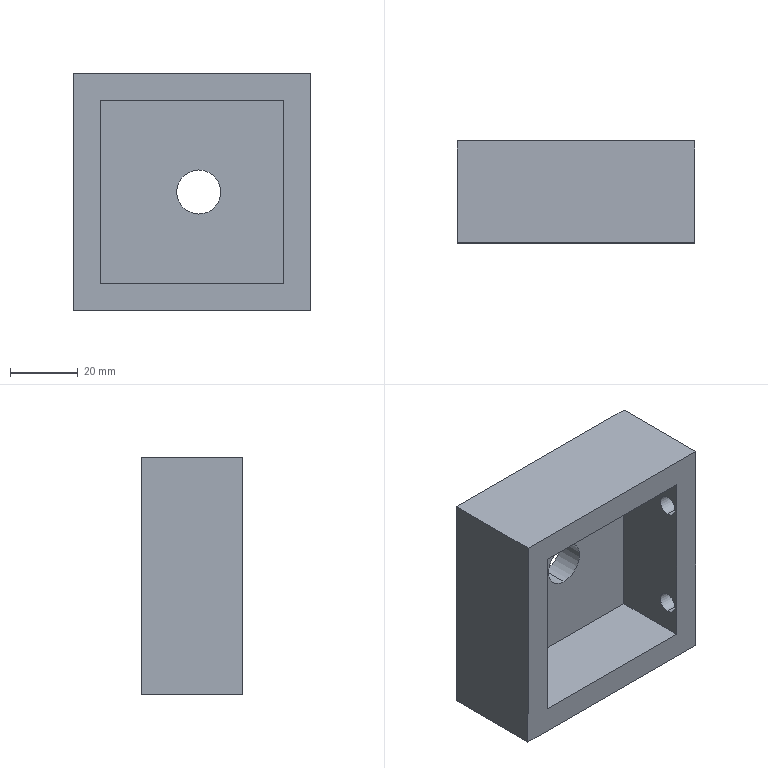Component | SolidWorks | GrippingMountingHousing-2 | 1 solid | 17 faces | box 70.08 x 30 x 70.08 mm | volume 81334 mm3 | plane 11 | cylinder 6 | commonest cylinder face diameters 6 x4 13 x2
build123d program:
from build123d import *

# Parameters (mm, degrees)
SKETCH1_2_W                   = 30
SKETCH1_2_H                   = 70
BOSS_EXTRUDE1_DEPTH           = 70
SHELL1_T                      = -8
SKETCH4_R                     = 3
CUT_EXTRUDE2_DEPTH            = 10
SKETCH1_R                     = 6.5
PISTON_ROD_THROUGH_HOLE_DEPTH = 8.5


with BuildPart() as part:
    # Sketch1_2 → Boss-Extrude1 (new body)
    with BuildSketch(Plane(origin=(0, 0, 0), x_dir=(1, 0, 0), z_dir=(0, 1, 0))):
        Rectangle(SKETCH1_2_W, SKETCH1_2_H)
    extrude(amount=BOSS_EXTRUDE1_DEPTH)

    # Shell1
    shell1_openings = [part.faces().sort_by_distance(p)[0] for p in [
        (15, 35, 0),
    ]]
    offset(amount=SHELL1_T, openings=shell1_openings, kind=Kind.INTERSECTION)

    # Sketch4 → Cut-Extrude2 (cut)
    with BuildSketch(Plane(origin=(0, 70, 0), x_dir=(1, 0, 0), z_dir=(0, 1, 0))):
        with Locations(Location((11.231, -17.525, 0), (0, 0, 270))):
            Circle(SKETCH4_R)
        with Locations(Location((11.231, 17.525, 0), (0, 0, 270))):
            Circle(SKETCH4_R)
    extrude(amount=-CUT_EXTRUDE2_DEPTH, mode=Mode.SUBTRACT)

    # Sketch1 → Piston Rod Through Hole (cut)
    with BuildSketch(Plane.ZY.offset(15)):
        with Locations((-0.0026, 37.002)):
            Circle(SKETCH1_R)
    extrude(amount=-PISTON_ROD_THROUGH_HOLE_DEPTH, mode=Mode.SUBTRACT)


solid = part.part

# Placed as in the assembly
solid = solid.moved(Location((-162.042, 776.54, 1109.793), (0, 0.0619, -90)))
STEP:
#1=COLOUR_RGB('',0.7922,0.8196,0.9333);
#2=FILL_AREA_STYLE_COLOUR('',#1);
#3=FILL_AREA_STYLE('',(#2));
#4=SURFACE_STYLE_FILL_AREA(#3);
#5=SURFACE_SIDE_STYLE('',(#4));
#6=SURFACE_STYLE_USAGE(.BOTH.,#5);
#7=PRESENTATION_STYLE_ASSIGNMENT((#6));
#8=CARTESIAN_POINT('',(-4.923,30.848,43.947));
#9=VERTEX_POINT('',#8);
#10=CARTESIAN_POINT('',(-4.923,30.848,43.435));
#11=VERTEX_POINT('',#10);
#12=CARTESIAN_POINT('',(-4.923,30.848,43.691));
#13=DIRECTION('',(0.,-1.,0.));
#14=DIRECTION('',(-0.00108,0.,-1.));
#15=AXIS2_PLACEMENT_3D('',#12,#13,#14);
#16=CIRCLE('',#15,0.2559);
#17=EDGE_CURVE('',#9,#11,#16,.T.);
#18=ORIENTED_EDGE('',*,*,#17,.T.);
#19=CARTESIAN_POINT('',(-4.923,31.163,43.435));
#20=VERTEX_POINT('',#19);
#21=CARTESIAN_POINT('',(-4.923,30.828,43.435));
#22=DIRECTION('',(-0.,1.,-0.));
#23=VECTOR('',#22,39.37);
#24=LINE('',#21,#23);
#25=EDGE_CURVE('',#11,#20,#24,.T.);
#26=ORIENTED_EDGE('',*,*,#25,.T.);
#27=CARTESIAN_POINT('',(-4.923,31.163,43.947));
#28=VERTEX_POINT('',#27);
#29=CARTESIAN_POINT('',(-4.923,31.163,43.691));
#30=DIRECTION('',(-0.,1.,-0.));
#31=DIRECTION('',(0.00108,0.,1.));
#32=AXIS2_PLACEMENT_3D('',#29,#30,#31);
#33=CIRCLE('',#32,0.2559);
#34=EDGE_CURVE('',#20,#28,#33,.T.);
#35=ORIENTED_EDGE('',*,*,#34,.T.);
#36=CARTESIAN_POINT('',(-4.923,30.828,43.947));
#37=DIRECTION('',(-0.,1.,-0.));
#38=VECTOR('',#37,39.37);
#39=LINE('',#36,#38);
#40=EDGE_CURVE('',#9,#28,#39,.T.);
#41=ORIENTED_EDGE('',*,*,#40,.F.);
#42=EDGE_LOOP('',(#18,#26,#35,#41));
#43=FACE_OUTER_BOUND('',#42,.T.);
#44=CARTESIAN_POINT('',(-4.923,30.828,43.691));
#45=DIRECTION('',(-0.,1.,-0.));
#46=DIRECTION('',(0.00108,0.,1.));
#47=AXIS2_PLACEMENT_3D('',#44,#45,#46);
#48=CYLINDRICAL_SURFACE('',#47,0.2559);
#49=ADVANCED_FACE('',(#43),#48,.F.);
#50=CARTESIAN_POINT('',(-3.938,30.13,44.498));
#51=VERTEX_POINT('',#50);
#52=CARTESIAN_POINT('',(-3.938,30.13,44.262));
#53=VERTEX_POINT('',#52);
#54=CARTESIAN_POINT('',(-3.938,30.13,44.38));
#55=DIRECTION('',(-1.,-0.,0.00108));
#56=DIRECTION('',(-0.00108,0.,-1.));
#57=AXIS2_PLACEMENT_3D('',#54,#55,#56);
#58=CIRCLE('',#57,0.1181);
#59=EDGE_CURVE('',#51,#53,#58,.T.);
#60=ORIENTED_EDGE('',*,*,#59,.T.);
#61=CARTESIAN_POINT('',(-3.623,30.13,44.261));
#62=VERTEX_POINT('',#61);
#63=CARTESIAN_POINT('',(-4.017,30.13,44.262));
#64=DIRECTION('',(1.,0.,-0.00108));
#65=VECTOR('',#64,39.37);
#66=LINE('',#63,#65);
#67=EDGE_CURVE('',#53,#62,#66,.T.);
#68=ORIENTED_EDGE('',*,*,#67,.T.);
#69=CARTESIAN_POINT('',(-3.623,30.13,44.498));
#70=VERTEX_POINT('',#69);
#71=CARTESIAN_POINT('',(-3.623,30.13,44.38));
#72=DIRECTION('',(1.,0.,-0.00108));
#73=DIRECTION('',(0.00108,0.,1.));
#74=AXIS2_PLACEMENT_3D('',#71,#72,#73);
#75=CIRCLE('',#74,0.1181);
#76=EDGE_CURVE('',#62,#70,#75,.T.);
#77=ORIENTED_EDGE('',*,*,#76,.T.);
#78=CARTESIAN_POINT('',(-4.017,30.13,44.498));
#79=DIRECTION('',(1.,0.,-0.00108));
#80=VECTOR('',#79,39.37);
#81=LINE('',#78,#80);
#82=EDGE_CURVE('',#51,#70,#81,.T.);
#83=ORIENTED_EDGE('',*,*,#82,.F.);
#84=EDGE_LOOP('',(#60,#68,#77,#83));
#85=FACE_OUTER_BOUND('',#84,.T.);
#86=CARTESIAN_POINT('',(-4.017,30.13,44.38));
#87=DIRECTION('',(1.,0.,-0.00108));
#88=DIRECTION('',(0.00108,0.,1.));
#89=AXIS2_PLACEMENT_3D('',#86,#87,#88);
#90=CYLINDRICAL_SURFACE('',#89,0.1181);
#91=ADVANCED_FACE('',(#85),#90,.F.);
#92=CARTESIAN_POINT('',(-3.939,30.13,43.118));
#93=VERTEX_POINT('',#92);
#94=CARTESIAN_POINT('',(-3.94,30.13,42.882));
#95=VERTEX_POINT('',#94);
#96=CARTESIAN_POINT('',(-3.939,30.13,43.));
#97=DIRECTION('',(-1.,-0.,0.00108));
#98=DIRECTION('',(-0.00108,0.,-1.));
#99=AXIS2_PLACEMENT_3D('',#96,#97,#98);
#100=CIRCLE('',#99,0.1181);
#101=EDGE_CURVE('',#93,#95,#100,.T.);
#102=ORIENTED_EDGE('',*,*,#101,.T.);
#103=CARTESIAN_POINT('',(-3.625,30.13,42.882));
#104=VERTEX_POINT('',#103);
#105=CARTESIAN_POINT('',(-4.018,30.13,42.882));
#106=DIRECTION('',(1.,0.,-0.00108));
#107=VECTOR('',#106,39.37);
#108=LINE('',#105,#107);
#109=EDGE_CURVE('',#95,#104,#108,.T.);
#110=ORIENTED_EDGE('',*,*,#109,.T.);
#111=CARTESIAN_POINT('',(-3.624,30.13,43.118));
#112=VERTEX_POINT('',#111);
#113=CARTESIAN_POINT('',(-3.624,30.13,43.));
#114=DIRECTION('',(1.,0.,-0.00108));
#115=DIRECTION('',(0.00108,0.,1.));
#116=AXIS2_PLACEMENT_3D('',#113,#114,#115);
#117=CIRCLE('',#116,0.1181);
#118=EDGE_CURVE('',#104,#112,#117,.T.);
#119=ORIENTED_EDGE('',*,*,#118,.T.);
#120=CARTESIAN_POINT('',(-4.018,30.13,43.118));
#121=DIRECTION('',(1.,0.,-0.00108));
#122=VECTOR('',#121,39.37);
#123=LINE('',#120,#122);
#124=EDGE_CURVE('',#93,#112,#123,.T.);
#125=ORIENTED_EDGE('',*,*,#124,.F.);
#126=EDGE_LOOP('',(#102,#110,#119,#125));
#127=FACE_OUTER_BOUND('',#126,.T.);
#128=CARTESIAN_POINT('',(-4.018,30.13,43.));
#129=DIRECTION('',(1.,0.,-0.00108));
#130=DIRECTION('',(0.00108,0.,1.));
#131=AXIS2_PLACEMENT_3D('',#128,#129,#130);
#132=CYLINDRICAL_SURFACE('',#131,0.1181);
#133=ADVANCED_FACE('',(#127),#132,.F.);
#134=CARTESIAN_POINT('',(-6.378,29.982,45.071));
#135=VERTEX_POINT('',#134);
#136=CARTESIAN_POINT('',(-6.381,29.982,42.315));
#137=VERTEX_POINT('',#136);
#138=CARTESIAN_POINT('',(-6.378,29.982,45.071));
#139=DIRECTION('',(-0.00108,-0.,-1.));
#140=VECTOR('',#139,39.37);
#141=LINE('',#138,#140);
#142=EDGE_CURVE('',#135,#137,#141,.T.);
#143=ORIENTED_EDGE('',*,*,#142,.T.);
#144=CARTESIAN_POINT('',(-3.625,29.982,42.312));
#145=VERTEX_POINT('',#144);
#146=CARTESIAN_POINT('',(-3.625,29.982,42.312));
#147=DIRECTION('',(-1.,-0.,0.00108));
#148=VECTOR('',#147,39.37);
#149=LINE('',#146,#148);
#150=EDGE_CURVE('',#145,#137,#149,.T.);
#151=ORIENTED_EDGE('',*,*,#150,.F.);
#152=CARTESIAN_POINT('',(-3.622,29.982,45.068));
#153=VERTEX_POINT('',#152);
#154=CARTESIAN_POINT('',(-3.622,29.982,45.068));
#155=DIRECTION('',(-0.00108,-0.,-1.));
#156=VECTOR('',#155,39.37);
#157=LINE('',#154,#156);
#158=EDGE_CURVE('',#153,#145,#157,.T.);
#159=ORIENTED_EDGE('',*,*,#158,.F.);
#160=CARTESIAN_POINT('',(-3.622,29.982,45.068));
#161=DIRECTION('',(-1.,-0.,0.00108));
#162=VECTOR('',#161,39.37);
#163=LINE('',#160,#162);
#164=EDGE_CURVE('',#153,#135,#163,.T.);
#165=ORIENTED_EDGE('',*,*,#164,.T.);
#166=EDGE_LOOP('',(#143,#151,#159,#165));
#167=FACE_OUTER_BOUND('',#166,.T.);
#168=CARTESIAN_POINT('',(-6.064,29.982,44.755));
#169=VERTEX_POINT('',#168);
#170=CARTESIAN_POINT('',(-6.066,29.982,42.629));
#171=VERTEX_POINT('',#170);
#172=CARTESIAN_POINT('',(-6.065,29.982,43.692));
#173=DIRECTION('',(-0.00108,-0.,-1.));
#174=VECTOR('',#173,39.37);
#175=LINE('',#172,#174);
#176=EDGE_CURVE('',#169,#171,#175,.T.);
#177=ORIENTED_EDGE('',*,*,#176,.F.);
#178=CARTESIAN_POINT('',(-3.938,29.982,44.753));
#179=VERTEX_POINT('',#178);
#180=CARTESIAN_POINT('',(-3.623,29.982,44.753));
#181=DIRECTION('',(-1.,-0.,0.00108));
#182=VECTOR('',#181,39.37);
#183=LINE('',#180,#182);
#184=EDGE_CURVE('',#179,#169,#183,.T.);
#185=ORIENTED_EDGE('',*,*,#184,.F.);
#186=CARTESIAN_POINT('',(-3.94,29.982,42.627));
#187=VERTEX_POINT('',#186);
#188=CARTESIAN_POINT('',(-3.939,29.982,43.69));
#189=DIRECTION('',(-0.00108,-0.,-1.));
#190=VECTOR('',#189,39.37);
#191=LINE('',#188,#190);
#192=EDGE_CURVE('',#179,#187,#191,.T.);
#193=ORIENTED_EDGE('',*,*,#192,.T.);
#194=CARTESIAN_POINT('',(-3.625,29.982,42.627));
#195=DIRECTION('',(-1.,-0.,0.00108));
#196=VECTOR('',#195,39.37);
#197=LINE('',#194,#196);
#198=EDGE_CURVE('',#187,#171,#197,.T.);
#199=ORIENTED_EDGE('',*,*,#198,.T.);
#200=EDGE_LOOP('',(#177,#185,#193,#199));
#201=FACE_BOUND('',#200,.T.);
#202=CARTESIAN_POINT('',(-3.622,29.982,45.068));
#203=DIRECTION('',(-0.,1.,-0.));
#204=DIRECTION('',(0.00108,0.,1.));
#205=AXIS2_PLACEMENT_3D('',#202,#203,#204);
#206=PLANE('',#205);
#207=ADVANCED_FACE('',(#167,#201),#206,.F.);
#208=CARTESIAN_POINT('',(-6.381,31.163,42.315));
#209=VERTEX_POINT('',#208);
#210=CARTESIAN_POINT('',(-6.381,31.163,42.315));
#211=DIRECTION('',(-0.,1.,-0.));
#212=VECTOR('',#211,39.37);
#213=LINE('',#210,#212);
#214=EDGE_CURVE('',#137,#209,#213,.T.);
#215=ORIENTED_EDGE('',*,*,#214,.T.);
#216=CARTESIAN_POINT('',(-3.625,31.163,42.312));
#217=VERTEX_POINT('',#216);
#218=CARTESIAN_POINT('',(-3.625,31.163,42.312));
#219=DIRECTION('',(-1.,-0.,0.00108));
#220=VECTOR('',#219,39.37);
#221=LINE('',#218,#220);
#222=EDGE_CURVE('',#217,#209,#221,.T.);
#223=ORIENTED_EDGE('',*,*,#222,.F.);
#224=CARTESIAN_POINT('',(-3.625,31.163,42.312));
#225=DIRECTION('',(-0.,1.,-0.));
#226=VECTOR('',#225,39.37);
#227=LINE('',#224,#226);
#228=EDGE_CURVE('',#145,#217,#227,.T.);
#229=ORIENTED_EDGE('',*,*,#228,.F.);
#230=ORIENTED_EDGE('',*,*,#150,.T.);
#231=EDGE_LOOP('',(#215,#223,#229,#230));
#232=FACE_OUTER_BOUND('',#231,.T.);
#233=CARTESIAN_POINT('',(-3.625,31.163,42.312));
#234=DIRECTION('',(0.00108,0.,1.));
#235=DIRECTION('',(0.,-1.,0.));
#236=AXIS2_PLACEMENT_3D('',#233,#234,#235);
#237=PLANE('',#236);
#238=ADVANCED_FACE('',(#232),#237,.F.);
#239=CARTESIAN_POINT('',(-4.923,31.163,43.691));
#240=DIRECTION('',(-0.,1.,-0.));
#241=DIRECTION('',(0.00108,0.,1.));
#242=AXIS2_PLACEMENT_3D('',#239,#240,#241);
#243=CIRCLE('',#242,0.2559);
#244=EDGE_CURVE('',#28,#20,#243,.T.);
#245=ORIENTED_EDGE('',*,*,#244,.F.);
#246=ORIENTED_EDGE('',*,*,#34,.F.);
#247=EDGE_LOOP('',(#245,#246));
#248=FACE_BOUND('',#247,.T.);
#249=CARTESIAN_POINT('',(-6.378,31.163,45.071));
#250=VERTEX_POINT('',#249);
#251=CARTESIAN_POINT('',(-6.378,31.163,45.071));
#252=DIRECTION('',(0.00108,0.,1.));
#253=VECTOR('',#252,39.37);
#254=LINE('',#251,#253);
#255=EDGE_CURVE('',#209,#250,#254,.T.);
#256=ORIENTED_EDGE('',*,*,#255,.T.);
#257=CARTESIAN_POINT('',(-3.622,31.163,45.068));
#258=VERTEX_POINT('',#257);
#259=CARTESIAN_POINT('',(-3.622,31.163,45.068));
#260=DIRECTION('',(-1.,-0.,0.00108));
#261=VECTOR('',#260,39.37);
#262=LINE('',#259,#261);
#263=EDGE_CURVE('',#258,#250,#262,.T.);
#264=ORIENTED_EDGE('',*,*,#263,.F.);
#265=CARTESIAN_POINT('',(-3.622,31.163,45.068));
#266=DIRECTION('',(0.00108,0.,1.));
#267=VECTOR('',#266,39.37);
#268=LINE('',#265,#267);
#269=EDGE_CURVE('',#217,#258,#268,.T.);
#270=ORIENTED_EDGE('',*,*,#269,.F.);
#271=ORIENTED_EDGE('',*,*,#222,.T.);
#272=EDGE_LOOP('',(#256,#264,#270,#271));
#273=FACE_OUTER_BOUND('',#272,.T.);
#274=CARTESIAN_POINT('',(-3.622,31.163,45.068));
#275=DIRECTION('',(0.,-1.,0.));
#276=DIRECTION('',(-0.00108,-0.,-1.));
#277=AXIS2_PLACEMENT_3D('',#274,#275,#276);
#278=PLANE('',#277);
#279=ADVANCED_FACE('',(#248,#273),#278,.F.);
#280=CARTESIAN_POINT('',(-6.378,31.163,45.071));
#281=DIRECTION('',(0.,-1.,0.));
#282=VECTOR('',#281,39.37);
#283=LINE('',#280,#282);
#284=EDGE_CURVE('',#250,#135,#283,.T.);
#285=ORIENTED_EDGE('',*,*,#284,.T.);
#286=ORIENTED_EDGE('',*,*,#164,.F.);
#287=CARTESIAN_POINT('',(-3.622,31.163,45.068));
#288=DIRECTION('',(0.,-1.,0.));
#289=VECTOR('',#288,39.37);
#290=LINE('',#287,#289);
#291=EDGE_CURVE('',#258,#153,#290,.T.);
#292=ORIENTED_EDGE('',*,*,#291,.F.);
#293=ORIENTED_EDGE('',*,*,#263,.T.);
#294=EDGE_LOOP('',(#285,#286,#292,#293));
#295=FACE_OUTER_BOUND('',#294,.T.);
#296=CARTESIAN_POINT('',(-3.622,31.163,45.068));
#297=DIRECTION('',(-0.00108,-0.,-1.));
#298=DIRECTION('',(-0.,1.,-0.));
#299=AXIS2_PLACEMENT_3D('',#296,#297,#298);
#300=PLANE('',#299);
#301=ADVANCED_FACE('',(#295),#300,.F.);
#302=CARTESIAN_POINT('',(-3.623,30.13,44.38));
#303=DIRECTION('',(1.,0.,-0.00108));
#304=DIRECTION('',(0.00108,0.,1.));
#305=AXIS2_PLACEMENT_3D('',#302,#303,#304);
#306=CIRCLE('',#305,0.1181);
#307=EDGE_CURVE('',#70,#62,#306,.T.);
#308=ORIENTED_EDGE('',*,*,#307,.F.);
#309=ORIENTED_EDGE('',*,*,#76,.F.);
#310=EDGE_LOOP('',(#308,#309));
#311=FACE_BOUND('',#310,.T.);
#312=CARTESIAN_POINT('',(-3.624,30.13,43.));
#313=DIRECTION('',(1.,0.,-0.00108));
#314=DIRECTION('',(0.00108,0.,1.));
#315=AXIS2_PLACEMENT_3D('',#312,#313,#314);
#316=CIRCLE('',#315,0.1181);
#317=EDGE_CURVE('',#112,#104,#316,.T.);
#318=ORIENTED_EDGE('',*,*,#317,.F.);
#319=ORIENTED_EDGE('',*,*,#118,.F.);
#320=EDGE_LOOP('',(#318,#319));
#321=FACE_BOUND('',#320,.T.);
#322=ORIENTED_EDGE('',*,*,#158,.T.);
#323=ORIENTED_EDGE('',*,*,#228,.T.);
#324=ORIENTED_EDGE('',*,*,#269,.T.);
#325=ORIENTED_EDGE('',*,*,#291,.T.);
#326=EDGE_LOOP('',(#322,#323,#324,#325));
#327=FACE_OUTER_BOUND('',#326,.T.);
#328=CARTESIAN_POINT('',(-3.624,30.572,43.69));
#329=DIRECTION('',(-1.,-0.,0.00108));
#330=DIRECTION('',(-0.00108,-0.,-1.));
#331=AXIS2_PLACEMENT_3D('',#328,#329,#330);
#332=PLANE('',#331);
#333=ADVANCED_FACE('',(#311,#321,#327),#332,.F.);
#334=ORIENTED_EDGE('',*,*,#142,.F.);
#335=ORIENTED_EDGE('',*,*,#284,.F.);
#336=ORIENTED_EDGE('',*,*,#255,.F.);
#337=ORIENTED_EDGE('',*,*,#214,.F.);
#338=EDGE_LOOP('',(#334,#335,#336,#337));
#339=FACE_OUTER_BOUND('',#338,.T.);
#340=CARTESIAN_POINT('',(-6.38,30.572,43.693));
#341=DIRECTION('',(-1.,-0.,0.00108));
#342=DIRECTION('',(-0.00108,-0.,-1.));
#343=AXIS2_PLACEMENT_3D('',#340,#341,#342);
#344=PLANE('',#343);
#345=ADVANCED_FACE('',(#339),#344,.T.);
#346=CARTESIAN_POINT('',(-6.066,30.848,42.629));
#347=VERTEX_POINT('',#346);
#348=CARTESIAN_POINT('',(-6.066,30.572,42.629));
#349=DIRECTION('',(-0.,1.,-0.));
#350=VECTOR('',#349,39.37);
#351=LINE('',#348,#350);
#352=EDGE_CURVE('',#171,#347,#351,.T.);
#353=ORIENTED_EDGE('',*,*,#352,.F.);
#354=ORIENTED_EDGE('',*,*,#198,.F.);
#355=CARTESIAN_POINT('',(-3.94,30.848,42.627));
#356=VERTEX_POINT('',#355);
#357=CARTESIAN_POINT('',(-3.94,30.572,42.627));
#358=DIRECTION('',(-0.,1.,-0.));
#359=VECTOR('',#358,39.37);
#360=LINE('',#357,#359);
#361=EDGE_CURVE('',#187,#356,#360,.T.);
#362=ORIENTED_EDGE('',*,*,#361,.T.);
#363=CARTESIAN_POINT('',(-3.625,30.848,42.627));
#364=DIRECTION('',(-1.,-0.,0.00108));
#365=VECTOR('',#364,39.37);
#366=LINE('',#363,#365);
#367=EDGE_CURVE('',#356,#347,#366,.T.);
#368=ORIENTED_EDGE('',*,*,#367,.T.);
#369=EDGE_LOOP('',(#353,#354,#362,#368));
#370=FACE_OUTER_BOUND('',#369,.T.);
#371=CARTESIAN_POINT('',(-3.625,31.163,42.627));
#372=DIRECTION('',(0.00108,0.,1.));
#373=DIRECTION('',(0.,-1.,0.));
#374=AXIS2_PLACEMENT_3D('',#371,#372,#373);
#375=PLANE('',#374);
#376=ADVANCED_FACE('',(#370),#375,.T.);
#377=ORIENTED_EDGE('',*,*,#17,.F.);
#378=CARTESIAN_POINT('',(-4.923,30.848,43.691));
#379=DIRECTION('',(0.,-1.,0.));
#380=DIRECTION('',(-0.00108,0.,-1.));
#381=AXIS2_PLACEMENT_3D('',#378,#379,#380);
#382=CIRCLE('',#381,0.2559);
#383=EDGE_CURVE('',#11,#9,#382,.T.);
#384=ORIENTED_EDGE('',*,*,#383,.F.);
#385=EDGE_LOOP('',(#377,#384));
#386=FACE_BOUND('',#385,.T.);
#387=CARTESIAN_POINT('',(-6.064,30.848,44.755));
#388=VERTEX_POINT('',#387);
#389=CARTESIAN_POINT('',(-6.065,30.848,43.692));
#390=DIRECTION('',(0.00108,0.,1.));
#391=VECTOR('',#390,39.37);
#392=LINE('',#389,#391);
#393=EDGE_CURVE('',#347,#388,#392,.T.);
#394=ORIENTED_EDGE('',*,*,#393,.F.);
#395=ORIENTED_EDGE('',*,*,#367,.F.);
#396=CARTESIAN_POINT('',(-3.938,30.848,44.753));
#397=VERTEX_POINT('',#396);
#398=CARTESIAN_POINT('',(-3.939,30.848,43.69));
#399=DIRECTION('',(0.00108,0.,1.));
#400=VECTOR('',#399,39.37);
#401=LINE('',#398,#400);
#402=EDGE_CURVE('',#356,#397,#401,.T.);
#403=ORIENTED_EDGE('',*,*,#402,.T.);
#404=CARTESIAN_POINT('',(-3.623,30.848,44.753));
#405=DIRECTION('',(-1.,-0.,0.00108));
#406=VECTOR('',#405,39.37);
#407=LINE('',#404,#406);
#408=EDGE_CURVE('',#397,#388,#407,.T.);
#409=ORIENTED_EDGE('',*,*,#408,.T.);
#410=EDGE_LOOP('',(#394,#395,#403,#409));
#411=FACE_OUTER_BOUND('',#410,.T.);
#412=CARTESIAN_POINT('',(-3.622,30.848,45.068));
#413=DIRECTION('',(0.,-1.,0.));
#414=DIRECTION('',(-0.00108,-0.,-1.));
#415=AXIS2_PLACEMENT_3D('',#412,#413,#414);
#416=PLANE('',#415);
#417=ADVANCED_FACE('',(#386,#411),#416,.T.);
#418=CARTESIAN_POINT('',(-6.064,30.572,44.755));
#419=DIRECTION('',(0.,-1.,0.));
#420=VECTOR('',#419,39.37);
#421=LINE('',#418,#420);
#422=EDGE_CURVE('',#388,#169,#421,.T.);
#423=ORIENTED_EDGE('',*,*,#422,.F.);
#424=ORIENTED_EDGE('',*,*,#408,.F.);
#425=CARTESIAN_POINT('',(-3.938,30.572,44.753));
#426=DIRECTION('',(0.,-1.,0.));
#427=VECTOR('',#426,39.37);
#428=LINE('',#425,#427);
#429=EDGE_CURVE('',#397,#179,#428,.T.);
#430=ORIENTED_EDGE('',*,*,#429,.T.);
#431=ORIENTED_EDGE('',*,*,#184,.T.);
#432=EDGE_LOOP('',(#423,#424,#430,#431));
#433=FACE_OUTER_BOUND('',#432,.T.);
#434=CARTESIAN_POINT('',(-3.623,31.163,44.753));
#435=DIRECTION('',(-0.00108,-0.,-1.));
#436=DIRECTION('',(-0.,1.,-0.));
#437=AXIS2_PLACEMENT_3D('',#434,#435,#436);
#438=PLANE('',#437);
#439=ADVANCED_FACE('',(#433),#438,.T.);
#440=ORIENTED_EDGE('',*,*,#59,.F.);
#441=CARTESIAN_POINT('',(-3.938,30.13,44.38));
#442=DIRECTION('',(-1.,-0.,0.00108));
#443=DIRECTION('',(-0.00108,0.,-1.));
#444=AXIS2_PLACEMENT_3D('',#441,#442,#443);
#445=CIRCLE('',#444,0.1181);
#446=EDGE_CURVE('',#53,#51,#445,.T.);
#447=ORIENTED_EDGE('',*,*,#446,.F.);
#448=EDGE_LOOP('',(#440,#447));
#449=FACE_BOUND('',#448,.T.);
#450=ORIENTED_EDGE('',*,*,#101,.F.);
#451=CARTESIAN_POINT('',(-3.939,30.13,43.));
#452=DIRECTION('',(-1.,-0.,0.00108));
#453=DIRECTION('',(-0.00108,0.,-1.));
#454=AXIS2_PLACEMENT_3D('',#451,#452,#453);
#455=CIRCLE('',#454,0.1181);
#456=EDGE_CURVE('',#95,#93,#455,.T.);
#457=ORIENTED_EDGE('',*,*,#456,.F.);
#458=EDGE_LOOP('',(#450,#457));
#459=FACE_BOUND('',#458,.T.);
#460=ORIENTED_EDGE('',*,*,#192,.F.);
#461=ORIENTED_EDGE('',*,*,#429,.F.);
#462=ORIENTED_EDGE('',*,*,#402,.F.);
#463=ORIENTED_EDGE('',*,*,#361,.F.);
#464=EDGE_LOOP('',(#460,#461,#462,#463));
#465=FACE_OUTER_BOUND('',#464,.T.);
#466=CARTESIAN_POINT('',(-3.939,30.572,43.69));
#467=DIRECTION('',(-1.,-0.,0.00108));
#468=DIRECTION('',(-0.00108,-0.,-1.));
#469=AXIS2_PLACEMENT_3D('',#466,#467,#468);
#470=PLANE('',#469);
#471=ADVANCED_FACE('',(#449,#459,#465),#470,.T.);
#472=ORIENTED_EDGE('',*,*,#176,.T.);
#473=ORIENTED_EDGE('',*,*,#352,.T.);
#474=ORIENTED_EDGE('',*,*,#393,.T.);
#475=ORIENTED_EDGE('',*,*,#422,.T.);
#476=EDGE_LOOP('',(#472,#473,#474,#475));
#477=FACE_OUTER_BOUND('',#476,.T.);
#478=CARTESIAN_POINT('',(-6.065,30.572,43.692));
#479=DIRECTION('',(-1.,-0.,0.00108));
#480=DIRECTION('',(-0.00108,-0.,-1.));
#481=AXIS2_PLACEMENT_3D('',#478,#479,#480);
#482=PLANE('',#481);
#483=ADVANCED_FACE('',(#477),#482,.F.);
#484=ORIENTED_EDGE('',*,*,#109,.F.);
#485=ORIENTED_EDGE('',*,*,#456,.T.);
#486=ORIENTED_EDGE('',*,*,#124,.T.);
#487=ORIENTED_EDGE('',*,*,#317,.T.);
#488=EDGE_LOOP('',(#484,#485,#486,#487));
#489=FACE_OUTER_BOUND('',#488,.T.);
#490=CARTESIAN_POINT('',(-4.018,30.13,43.));
#491=DIRECTION('',(1.,0.,-0.00108));
#492=DIRECTION('',(0.00108,0.,1.));
#493=AXIS2_PLACEMENT_3D('',#490,#491,#492);
#494=CYLINDRICAL_SURFACE('',#493,0.1181);
#495=ADVANCED_FACE('',(#489),#494,.F.);
#496=ORIENTED_EDGE('',*,*,#67,.F.);
#497=ORIENTED_EDGE('',*,*,#446,.T.);
#498=ORIENTED_EDGE('',*,*,#82,.T.);
#499=ORIENTED_EDGE('',*,*,#307,.T.);
#500=EDGE_LOOP('',(#496,#497,#498,#499));
#501=FACE_OUTER_BOUND('',#500,.T.);
#502=CARTESIAN_POINT('',(-4.017,30.13,44.38));
#503=DIRECTION('',(1.,0.,-0.00108));
#504=DIRECTION('',(0.00108,0.,1.));
#505=AXIS2_PLACEMENT_3D('',#502,#503,#504);
#506=CYLINDRICAL_SURFACE('',#505,0.1181);
#507=ADVANCED_FACE('',(#501),#506,.F.);
#508=ORIENTED_EDGE('',*,*,#25,.F.);
#509=ORIENTED_EDGE('',*,*,#383,.T.);
#510=ORIENTED_EDGE('',*,*,#40,.T.);
#511=ORIENTED_EDGE('',*,*,#244,.T.);
#512=EDGE_LOOP('',(#508,#509,#510,#511));
#513=FACE_OUTER_BOUND('',#512,.T.);
#514=CARTESIAN_POINT('',(-4.923,30.828,43.691));
#515=DIRECTION('',(-0.,1.,-0.));
#516=DIRECTION('',(0.00108,0.,1.));
#517=AXIS2_PLACEMENT_3D('',#514,#515,#516);
#518=CYLINDRICAL_SURFACE('',#517,0.2559);
#519=ADVANCED_FACE('',(#513),#518,.F.);
#520=CLOSED_SHELL('',(#49,#91,#133,#207,#238,#279,#301,#333,#345,#376,#417,#439,#471,#483,#495,#507,#519));
#521=MANIFOLD_SOLID_BREP('',#520);
#522=STYLED_ITEM('',(#7),#521);
#523=(LENGTH_UNIT()NAMED_UNIT(*)SI_UNIT($,.METRE.));
#524=LENGTH_MEASURE_WITH_UNIT(LENGTH_MEASURE(0.0254),#523);
#525=DIMENSIONAL_EXPONENTS(1.,0.,0.,0.,0.,0.,0.);
#526=(CONVERSION_BASED_UNIT('',#524)LENGTH_UNIT()NAMED_UNIT(#525));
#527=UNCERTAINTY_MEASURE_WITH_UNIT(LENGTH_MEASURE(0.00001),#526,'','');
#528=(NAMED_UNIT(*)PLANE_ANGLE_UNIT()SI_UNIT($,.RADIAN.));
#529=(NAMED_UNIT(*)SI_UNIT($,.STERADIAN.)SOLID_ANGLE_UNIT());
#530=(GEOMETRIC_REPRESENTATION_CONTEXT(3)GLOBAL_UNCERTAINTY_ASSIGNED_CONTEXT((#527))GLOBAL_UNIT_ASSIGNED_CONTEXT((#526,#528,#529))REPRESENTATION_CONTEXT('',''));
#531=MECHANICAL_DESIGN_GEOMETRIC_PRESENTATION_REPRESENTATION('',(#522),#530);
#532=CARTESIAN_POINT('',(0.,0.,0.));
#533=DIRECTION('',(0.,0.,1.));
#534=DIRECTION('',(1.,0.,0.));
#535=AXIS2_PLACEMENT_3D('',#532,#533,#534);
#536=(LENGTH_UNIT()NAMED_UNIT(*)SI_UNIT($,.METRE.));
#537=LENGTH_MEASURE_WITH_UNIT(LENGTH_MEASURE(0.0254),#536);
#538=DIMENSIONAL_EXPONENTS(1.,0.,0.,0.,0.,0.,0.);
#539=(CONVERSION_BASED_UNIT('',#537)LENGTH_UNIT()NAMED_UNIT(#538));
#540=UNCERTAINTY_MEASURE_WITH_UNIT(LENGTH_MEASURE(0.00001),#539,'','');
#541=(NAMED_UNIT(*)PLANE_ANGLE_UNIT()SI_UNIT($,.RADIAN.));
#542=(NAMED_UNIT(*)SI_UNIT($,.STERADIAN.)SOLID_ANGLE_UNIT());
#543=(GEOMETRIC_REPRESENTATION_CONTEXT(3)GLOBAL_UNCERTAINTY_ASSIGNED_CONTEXT((#540))GLOBAL_UNIT_ASSIGNED_CONTEXT((#539,#541,#542))REPRESENTATION_CONTEXT('',''));
#544=ADVANCED_BREP_SHAPE_REPRESENTATION('',(#521,#535),#543);
#545=PRESENTATION_LAYER_ASSIGNMENT('','',(#522));